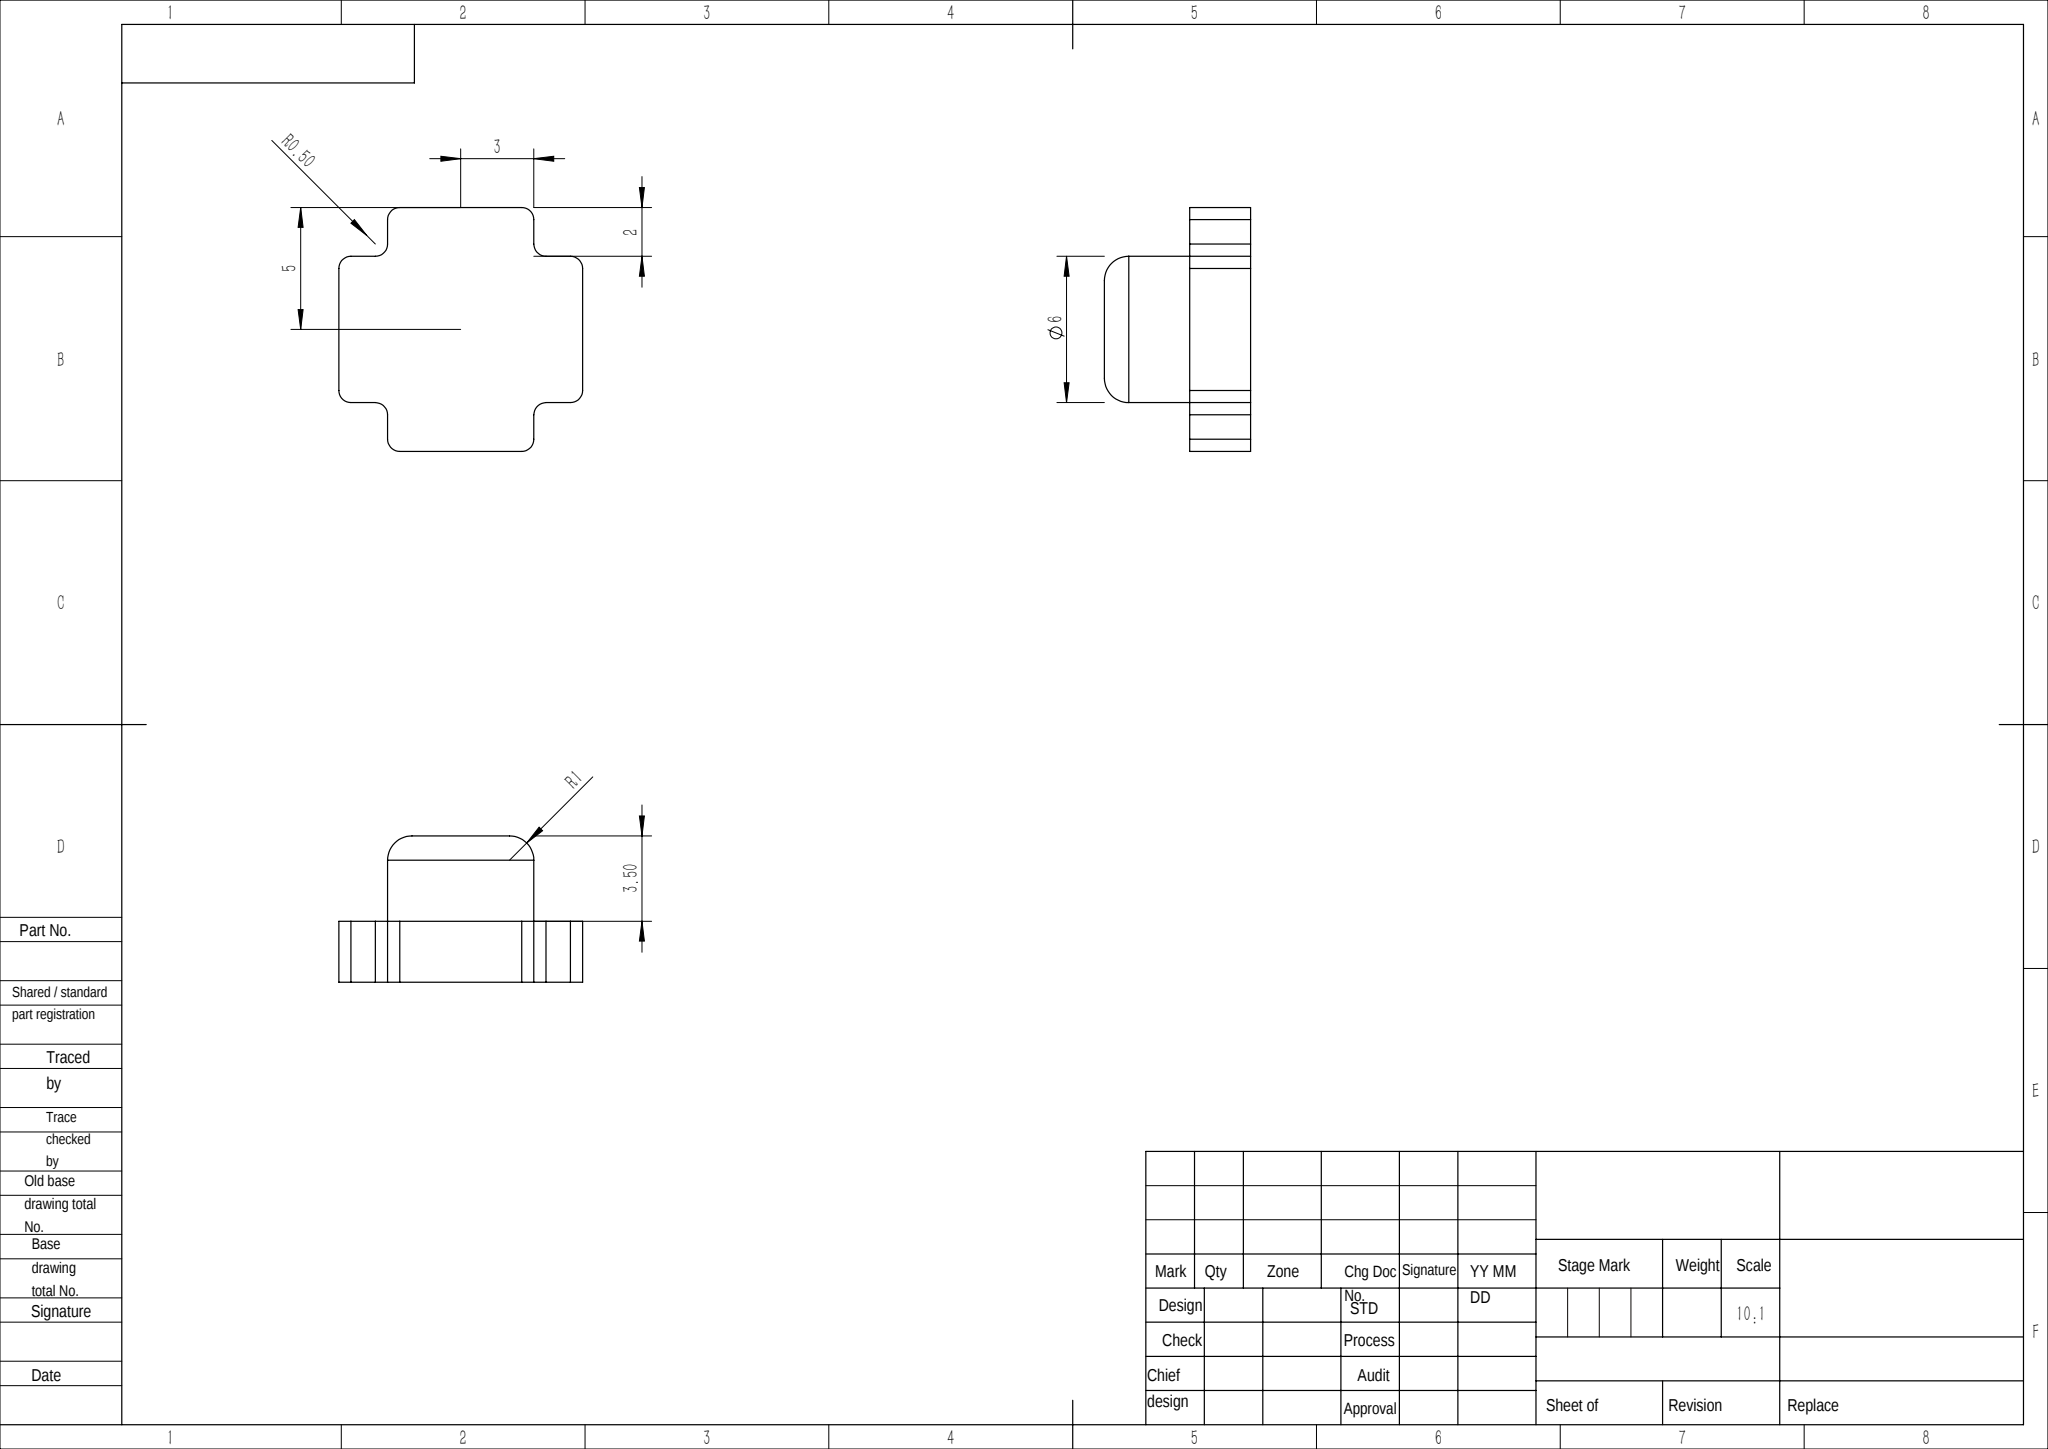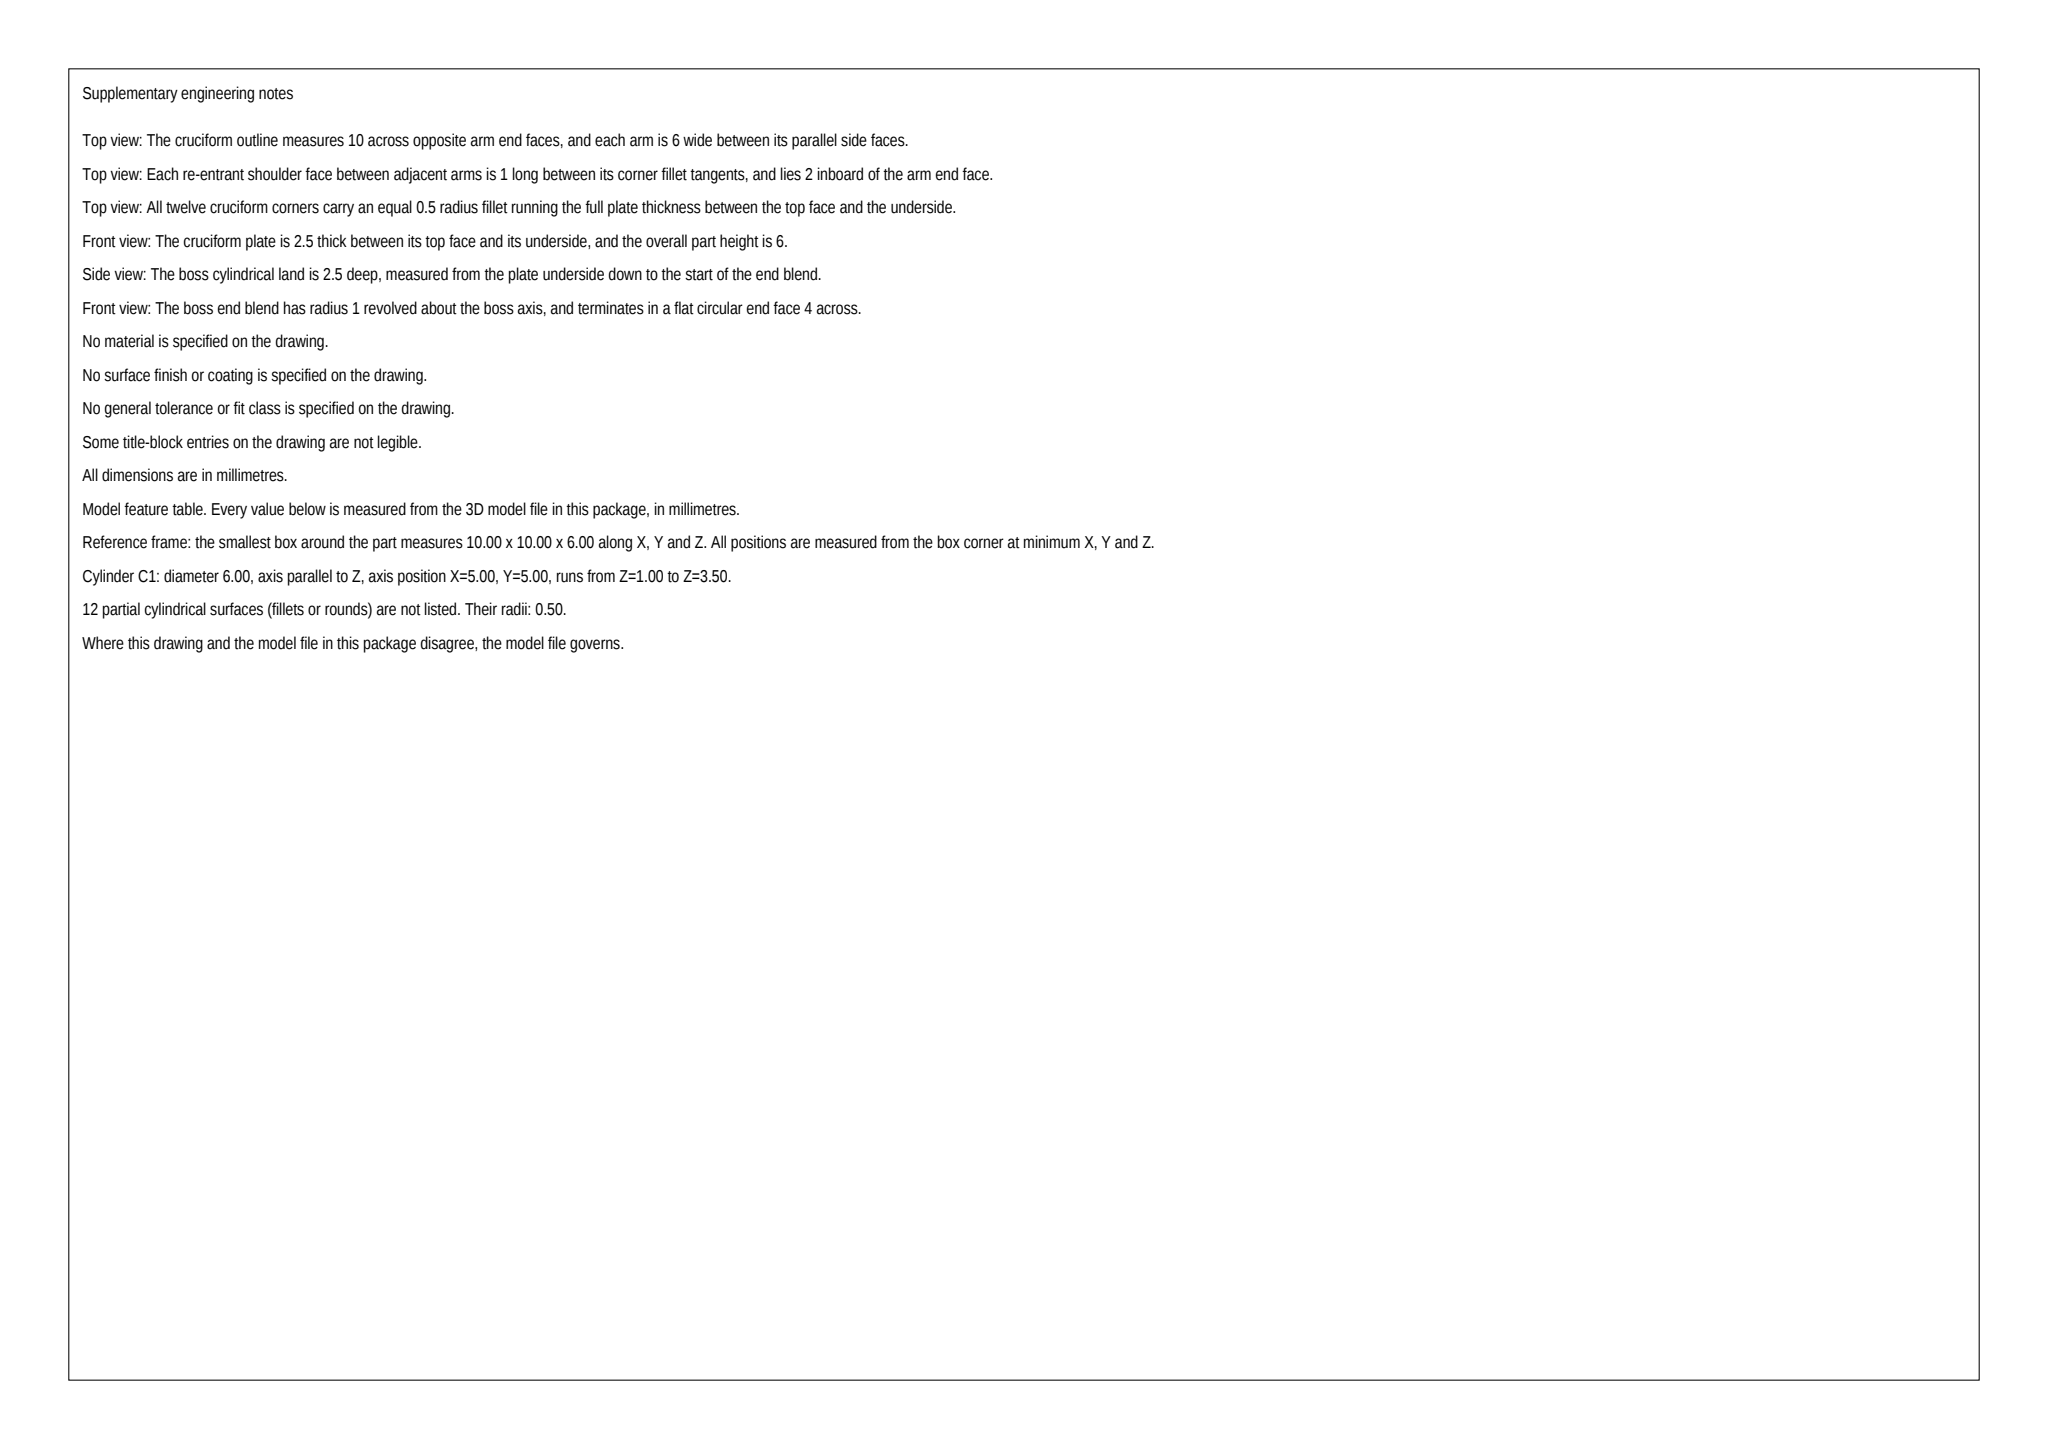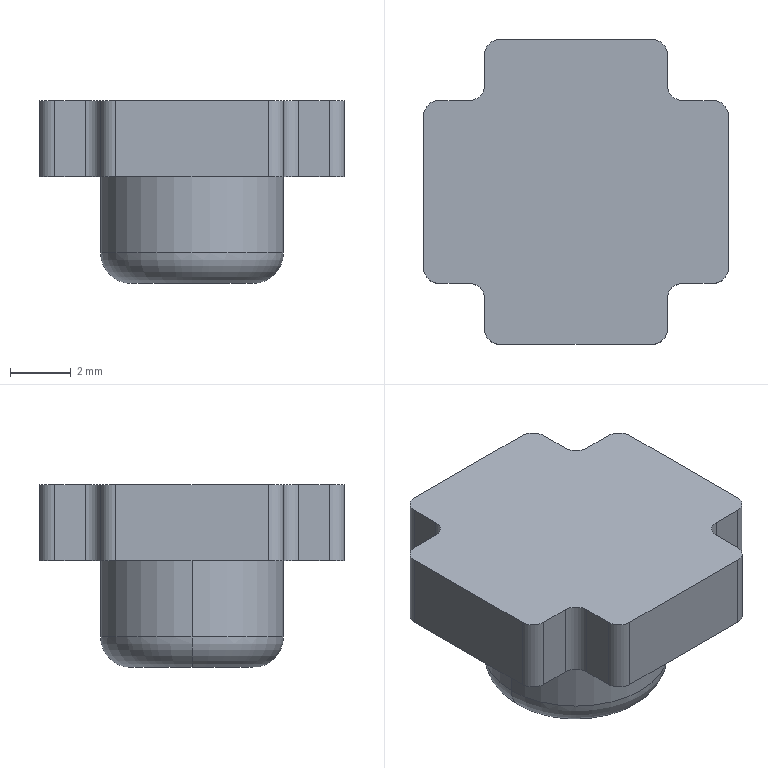Part | SolidWorks | mm | 1 solid | 31 faces | box 10 x 10 x 6 mm | volume 305 mm3 | plane 15 | cylinder 14 | torus 2 | commonest cylinder face diameters 1 x12 6 x2
Drawing notes:
Ø6 BOSS CONCENTRIC W/ 10x10 CROSS, 5 FROM EACH OUTER EDGE | from the solid: cyl dia 6 axis z at (5,5) in 10x10 bbox; outer planes x/y 0 & 10
R0.50 TYP 12 PLCS, ALL CROSS CORNERS | from the solid: 12 x cyl dia 1.0 (R0.5) axis z, len 2.5, at cross corner positions
UNSPECIFIED FILLETS R1 | from the solid: fillet_radii [[1.0, 2]] on Ø6 boss top edge
OVERALL HT 6 (2.50 BASE + 3.50 BOSS) | from the solid: bbox_xyz z = 6.0; z planes 0.0, 3.5, 6.0
build123d program:
from build123d import *

# Parameters (mm, degrees)
SKETCH1_R           = 3
BOSS_EXTRUDE1_DEPTH = 3.5
BOSS_EXTRUDE2_DEPTH = 2.5
FILLET1_R           = 1
FILLET2_R           = 0.5


with BuildPart() as part:
    # Sketch1 → Boss-Extrude1 (new body)
    with BuildSketch(Plane.XY):
        Circle(SKETCH1_R)
    extrude(amount=BOSS_EXTRUDE1_DEPTH)

    # Sketch2 → Boss-Extrude2 (add)
    with BuildSketch(Plane.XY.offset(3.5)):
        Polygon((-3, 5), (3, 5), (3, 3), (5, 3), (5, -3), (3, -3), (3, -5), (-3, -5), (-3, -3), (-5, -3), (-5, 3), (-3, 3), align=None)
    extrude(amount=BOSS_EXTRUDE2_DEPTH)

    # Fillet1
    fillet1_edges = [part.edges().sort_by_distance(p)[0] for p in [
        (-3, 0, 0),
    ]]
    fillet(fillet1_edges, radius=FILLET1_R)

    # Fillet2
    fillet2_edges = [part.edges().sort_by_distance(p)[0] for p in [
        (5, -3, 4.75),
        (5, 3, 4.75),
        (3, 3, 4.75),
        (3, 5, 4.75),
        (-3, 5, 4.75),
        (-3, 3, 4.75),
        (-5, 3, 4.75),
        (-5, -3, 4.75),
        (-3, -3, 4.75),
        (-3, -5, 4.75),
        (3, -5, 4.75),
        (3, -3, 4.75),
    ]]
    fillet(fillet2_edges, radius=FILLET2_R)


solid = part.part